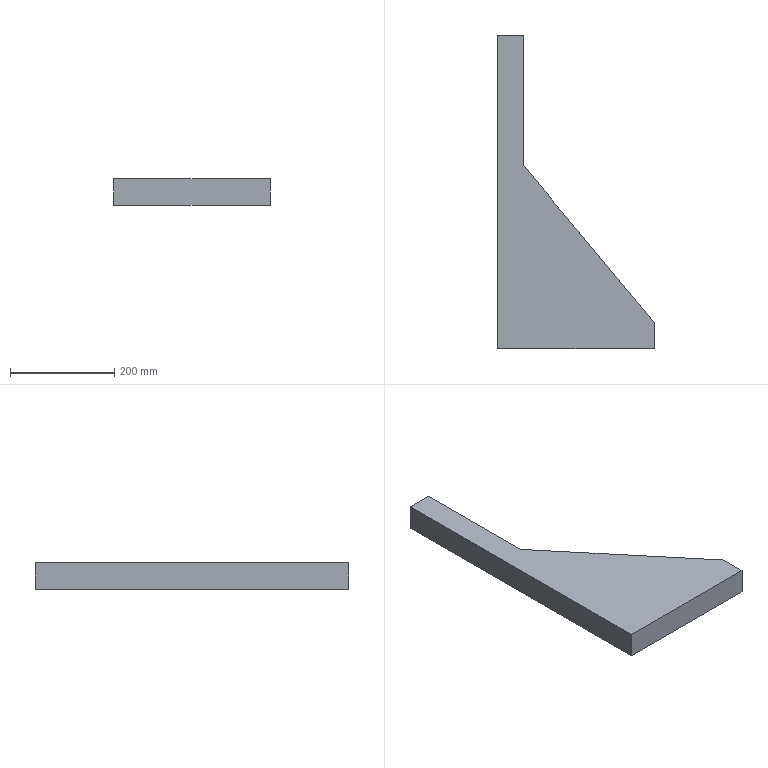Component | SolidWorks | ST60-07-2 | 1 solid | 8 faces | box 300 x 600 x 50 mm | volume 4000000 mm3 | plane 8
build123d program:
from build123d import *

# Parameters (mm, degrees)
BOSS_EXTRUDE1_DEPTH = 50


with BuildPart() as part:
    # Sketch1 → Boss-Extrude1 (new body)
    with BuildSketch(Plane.XY):
        Polygon((0, 300), (0, 0), (600, 0), (600, 50), (350, 50), (50, 300), align=None)
    extrude(amount=BOSS_EXTRUDE1_DEPTH)


solid = part.part

# Placed as in the assembly
solid = solid.moved(Location((277.993, 135.454, -1551.4), (180, 0, -90)))
STEP:
#1=COLOUR_RGB('',0.7922,0.8196,0.9333);
#2=FILL_AREA_STYLE_COLOUR('',#1);
#3=FILL_AREA_STYLE('',(#2));
#4=SURFACE_STYLE_FILL_AREA(#3);
#5=SURFACE_SIDE_STYLE('',(#4));
#6=SURFACE_STYLE_USAGE(.BOTH.,#5);
#7=PRESENTATION_STYLE_ASSIGNMENT((#6));
#8=CARTESIAN_POINT('',(22.756,7.301,-61.079));
#9=VERTEX_POINT('',#8);
#10=CARTESIAN_POINT('',(22.756,5.333,-61.079));
#11=VERTEX_POINT('',#10);
#12=CARTESIAN_POINT('',(22.756,7.301,-61.079));
#13=DIRECTION('',(0.,-1.,0.));
#14=VECTOR('',#13,39.37);
#15=LINE('',#12,#14);
#16=EDGE_CURVE('',#9,#11,#15,.T.);
#17=ORIENTED_EDGE('',*,*,#16,.T.);
#18=CARTESIAN_POINT('',(22.756,5.333,-63.047));
#19=VERTEX_POINT('',#18);
#20=CARTESIAN_POINT('',(22.756,5.333,-63.047));
#21=DIRECTION('',(0.,0.,1.));
#22=VECTOR('',#21,39.37);
#23=LINE('',#20,#22);
#24=EDGE_CURVE('',#19,#11,#23,.T.);
#25=ORIENTED_EDGE('',*,*,#24,.F.);
#26=CARTESIAN_POINT('',(22.756,7.301,-63.047));
#27=VERTEX_POINT('',#26);
#28=CARTESIAN_POINT('',(22.756,7.301,-63.047));
#29=DIRECTION('',(0.,-1.,0.));
#30=VECTOR('',#29,39.37);
#31=LINE('',#28,#30);
#32=EDGE_CURVE('',#27,#19,#31,.T.);
#33=ORIENTED_EDGE('',*,*,#32,.F.);
#34=CARTESIAN_POINT('',(22.756,7.301,-63.047));
#35=DIRECTION('',(0.,0.,1.));
#36=VECTOR('',#35,39.37);
#37=LINE('',#34,#36);
#38=EDGE_CURVE('',#27,#9,#37,.T.);
#39=ORIENTED_EDGE('',*,*,#38,.T.);
#40=EDGE_LOOP('',(#17,#25,#33,#39));
#41=FACE_OUTER_BOUND('',#40,.T.);
#42=CARTESIAN_POINT('',(22.756,7.301,-63.047));
#43=DIRECTION('',(-1.,-0.,0.));
#44=DIRECTION('',(0.,0.,1.));
#45=AXIS2_PLACEMENT_3D('',#42,#43,#44);
#46=PLANE('',#45);
#47=ADVANCED_FACE('',(#41),#46,.F.);
#48=CARTESIAN_POINT('',(10.945,5.333,-61.079));
#49=VERTEX_POINT('',#48);
#50=CARTESIAN_POINT('',(22.756,5.333,-61.079));
#51=DIRECTION('',(-1.,-0.,0.));
#52=VECTOR('',#51,39.37);
#53=LINE('',#50,#52);
#54=EDGE_CURVE('',#11,#49,#53,.T.);
#55=ORIENTED_EDGE('',*,*,#54,.T.);
#56=CARTESIAN_POINT('',(10.945,5.333,-63.047));
#57=VERTEX_POINT('',#56);
#58=CARTESIAN_POINT('',(10.945,5.333,-63.047));
#59=DIRECTION('',(0.,0.,1.));
#60=VECTOR('',#59,39.37);
#61=LINE('',#58,#60);
#62=EDGE_CURVE('',#57,#49,#61,.T.);
#63=ORIENTED_EDGE('',*,*,#62,.F.);
#64=CARTESIAN_POINT('',(22.756,5.333,-63.047));
#65=DIRECTION('',(-1.,-0.,0.));
#66=VECTOR('',#65,39.37);
#67=LINE('',#64,#66);
#68=EDGE_CURVE('',#19,#57,#67,.T.);
#69=ORIENTED_EDGE('',*,*,#68,.F.);
#70=ORIENTED_EDGE('',*,*,#24,.T.);
#71=EDGE_LOOP('',(#55,#63,#69,#70));
#72=FACE_OUTER_BOUND('',#71,.T.);
#73=CARTESIAN_POINT('',(22.756,5.333,-63.047));
#74=DIRECTION('',(-0.,1.,-0.));
#75=DIRECTION('',(1.,0.,-0.));
#76=AXIS2_PLACEMENT_3D('',#73,#74,#75);
#77=PLANE('',#76);
#78=ADVANCED_FACE('',(#72),#77,.F.);
#79=CARTESIAN_POINT('',(10.945,28.955,-61.079));
#80=VERTEX_POINT('',#79);
#81=CARTESIAN_POINT('',(10.945,5.333,-61.079));
#82=DIRECTION('',(-0.,1.,-0.));
#83=VECTOR('',#82,39.37);
#84=LINE('',#81,#83);
#85=EDGE_CURVE('',#49,#80,#84,.T.);
#86=ORIENTED_EDGE('',*,*,#85,.T.);
#87=CARTESIAN_POINT('',(10.945,28.955,-63.047));
#88=VERTEX_POINT('',#87);
#89=CARTESIAN_POINT('',(10.945,28.955,-63.047));
#90=DIRECTION('',(0.,0.,1.));
#91=VECTOR('',#90,39.37);
#92=LINE('',#89,#91);
#93=EDGE_CURVE('',#88,#80,#92,.T.);
#94=ORIENTED_EDGE('',*,*,#93,.F.);
#95=CARTESIAN_POINT('',(10.945,5.333,-63.047));
#96=DIRECTION('',(-0.,1.,-0.));
#97=VECTOR('',#96,39.37);
#98=LINE('',#95,#97);
#99=EDGE_CURVE('',#57,#88,#98,.T.);
#100=ORIENTED_EDGE('',*,*,#99,.F.);
#101=ORIENTED_EDGE('',*,*,#62,.T.);
#102=EDGE_LOOP('',(#86,#94,#100,#101));
#103=FACE_OUTER_BOUND('',#102,.T.);
#104=CARTESIAN_POINT('',(10.945,5.333,-63.047));
#105=DIRECTION('',(1.,0.,-0.));
#106=DIRECTION('',(-0.,-0.,-1.));
#107=AXIS2_PLACEMENT_3D('',#104,#105,#106);
#108=PLANE('',#107);
#109=ADVANCED_FACE('',(#103),#108,.F.);
#110=CARTESIAN_POINT('',(12.913,28.955,-61.079));
#111=VERTEX_POINT('',#110);
#112=CARTESIAN_POINT('',(10.945,28.955,-61.079));
#113=DIRECTION('',(1.,0.,-0.));
#114=VECTOR('',#113,39.37);
#115=LINE('',#112,#114);
#116=EDGE_CURVE('',#80,#111,#115,.T.);
#117=ORIENTED_EDGE('',*,*,#116,.T.);
#118=CARTESIAN_POINT('',(12.913,28.955,-63.047));
#119=VERTEX_POINT('',#118);
#120=CARTESIAN_POINT('',(12.913,28.955,-63.047));
#121=DIRECTION('',(0.,0.,1.));
#122=VECTOR('',#121,39.37);
#123=LINE('',#120,#122);
#124=EDGE_CURVE('',#119,#111,#123,.T.);
#125=ORIENTED_EDGE('',*,*,#124,.F.);
#126=CARTESIAN_POINT('',(10.945,28.955,-63.047));
#127=DIRECTION('',(1.,0.,-0.));
#128=VECTOR('',#127,39.37);
#129=LINE('',#126,#128);
#130=EDGE_CURVE('',#88,#119,#129,.T.);
#131=ORIENTED_EDGE('',*,*,#130,.F.);
#132=ORIENTED_EDGE('',*,*,#93,.T.);
#133=EDGE_LOOP('',(#117,#125,#131,#132));
#134=FACE_OUTER_BOUND('',#133,.T.);
#135=CARTESIAN_POINT('',(10.945,28.955,-63.047));
#136=DIRECTION('',(0.,-1.,0.));
#137=DIRECTION('',(-0.,-0.,-1.));
#138=AXIS2_PLACEMENT_3D('',#135,#136,#137);
#139=PLANE('',#138);
#140=ADVANCED_FACE('',(#134),#139,.F.);
#141=CARTESIAN_POINT('',(12.913,19.112,-61.079));
#142=VERTEX_POINT('',#141);
#143=CARTESIAN_POINT('',(12.913,28.955,-61.079));
#144=DIRECTION('',(-0.,-1.,0.));
#145=VECTOR('',#144,39.37);
#146=LINE('',#143,#145);
#147=EDGE_CURVE('',#111,#142,#146,.T.);
#148=ORIENTED_EDGE('',*,*,#147,.T.);
#149=CARTESIAN_POINT('',(12.913,19.112,-63.047));
#150=VERTEX_POINT('',#149);
#151=CARTESIAN_POINT('',(12.913,19.112,-63.047));
#152=DIRECTION('',(0.,0.,1.));
#153=VECTOR('',#152,39.37);
#154=LINE('',#151,#153);
#155=EDGE_CURVE('',#150,#142,#154,.T.);
#156=ORIENTED_EDGE('',*,*,#155,.F.);
#157=CARTESIAN_POINT('',(12.913,28.955,-63.047));
#158=DIRECTION('',(-0.,-1.,0.));
#159=VECTOR('',#158,39.37);
#160=LINE('',#157,#159);
#161=EDGE_CURVE('',#119,#150,#160,.T.);
#162=ORIENTED_EDGE('',*,*,#161,.F.);
#163=ORIENTED_EDGE('',*,*,#124,.T.);
#164=EDGE_LOOP('',(#148,#156,#162,#163));
#165=FACE_OUTER_BOUND('',#164,.T.);
#166=CARTESIAN_POINT('',(12.913,28.955,-63.047));
#167=DIRECTION('',(-1.,0.,0.));
#168=DIRECTION('',(0.,1.,-0.));
#169=AXIS2_PLACEMENT_3D('',#166,#167,#168);
#170=PLANE('',#169);
#171=ADVANCED_FACE('',(#165),#170,.F.);
#172=CARTESIAN_POINT('',(12.913,19.112,-61.079));
#173=DIRECTION('',(0.6402,-0.7682,-0.));
#174=VECTOR('',#173,39.37);
#175=LINE('',#172,#174);
#176=EDGE_CURVE('',#142,#9,#175,.T.);
#177=ORIENTED_EDGE('',*,*,#176,.T.);
#178=ORIENTED_EDGE('',*,*,#38,.F.);
#179=CARTESIAN_POINT('',(12.913,19.112,-63.047));
#180=DIRECTION('',(0.6402,-0.7682,-0.));
#181=VECTOR('',#180,39.37);
#182=LINE('',#179,#181);
#183=EDGE_CURVE('',#150,#27,#182,.T.);
#184=ORIENTED_EDGE('',*,*,#183,.F.);
#185=ORIENTED_EDGE('',*,*,#155,.T.);
#186=EDGE_LOOP('',(#177,#178,#184,#185));
#187=FACE_OUTER_BOUND('',#186,.T.);
#188=CARTESIAN_POINT('',(12.913,19.112,-63.047));
#189=DIRECTION('',(-0.7682,-0.6402,0.));
#190=DIRECTION('',(-0.6402,0.7682,0.));
#191=AXIS2_PLACEMENT_3D('',#188,#189,#190);
#192=PLANE('',#191);
#193=ADVANCED_FACE('',(#187),#192,.F.);
#194=ORIENTED_EDGE('',*,*,#32,.T.);
#195=ORIENTED_EDGE('',*,*,#68,.T.);
#196=ORIENTED_EDGE('',*,*,#99,.T.);
#197=ORIENTED_EDGE('',*,*,#130,.T.);
#198=ORIENTED_EDGE('',*,*,#161,.T.);
#199=ORIENTED_EDGE('',*,*,#183,.T.);
#200=EDGE_LOOP('',(#194,#195,#196,#197,#198,#199));
#201=FACE_OUTER_BOUND('',#200,.T.);
#202=CARTESIAN_POINT('',(10.945,5.333,-63.047));
#203=DIRECTION('',(-0.,-0.,-1.));
#204=DIRECTION('',(-0.,1.,-0.));
#205=AXIS2_PLACEMENT_3D('',#202,#203,#204);
#206=PLANE('',#205);
#207=ADVANCED_FACE('',(#201),#206,.T.);
#208=ORIENTED_EDGE('',*,*,#16,.F.);
#209=ORIENTED_EDGE('',*,*,#176,.F.);
#210=ORIENTED_EDGE('',*,*,#147,.F.);
#211=ORIENTED_EDGE('',*,*,#116,.F.);
#212=ORIENTED_EDGE('',*,*,#85,.F.);
#213=ORIENTED_EDGE('',*,*,#54,.F.);
#214=EDGE_LOOP('',(#208,#209,#210,#211,#212,#213));
#215=FACE_OUTER_BOUND('',#214,.T.);
#216=CARTESIAN_POINT('',(10.945,5.333,-61.079));
#217=DIRECTION('',(-0.,-0.,-1.));
#218=DIRECTION('',(-0.,1.,-0.));
#219=AXIS2_PLACEMENT_3D('',#216,#217,#218);
#220=PLANE('',#219);
#221=ADVANCED_FACE('',(#215),#220,.F.);
#222=CLOSED_SHELL('',(#47,#78,#109,#140,#171,#193,#207,#221));
#223=MANIFOLD_SOLID_BREP('',#222);
#224=STYLED_ITEM('',(#7),#223);
#225=(LENGTH_UNIT()NAMED_UNIT(*)SI_UNIT($,.METRE.));
#226=LENGTH_MEASURE_WITH_UNIT(LENGTH_MEASURE(0.0254),#225);
#227=DIMENSIONAL_EXPONENTS(1.,0.,0.,0.,0.,0.,0.);
#228=(CONVERSION_BASED_UNIT('',#226)LENGTH_UNIT()NAMED_UNIT(#227));
#229=UNCERTAINTY_MEASURE_WITH_UNIT(LENGTH_MEASURE(0.00001),#228,'','');
#230=(NAMED_UNIT(*)PLANE_ANGLE_UNIT()SI_UNIT($,.RADIAN.));
#231=(NAMED_UNIT(*)SI_UNIT($,.STERADIAN.)SOLID_ANGLE_UNIT());
#232=(GEOMETRIC_REPRESENTATION_CONTEXT(3)GLOBAL_UNCERTAINTY_ASSIGNED_CONTEXT((#229))GLOBAL_UNIT_ASSIGNED_CONTEXT((#228,#230,#231))REPRESENTATION_CONTEXT('',''));
#233=MECHANICAL_DESIGN_GEOMETRIC_PRESENTATION_REPRESENTATION('',(#224),#232);
#234=PRESENTATION_LAYER_ASSIGNMENT('','',(#224));
#235=CARTESIAN_POINT('',(0.,0.,0.));
#236=DIRECTION('',(0.,0.,1.));
#237=DIRECTION('',(1.,0.,0.));
#238=AXIS2_PLACEMENT_3D('',#235,#236,#237);
#239=(LENGTH_UNIT()NAMED_UNIT(*)SI_UNIT($,.METRE.));
#240=LENGTH_MEASURE_WITH_UNIT(LENGTH_MEASURE(0.0254),#239);
#241=DIMENSIONAL_EXPONENTS(1.,0.,0.,0.,0.,0.,0.);
#242=(CONVERSION_BASED_UNIT('',#240)LENGTH_UNIT()NAMED_UNIT(#241));
#243=UNCERTAINTY_MEASURE_WITH_UNIT(LENGTH_MEASURE(0.00001),#242,'','');
#244=(NAMED_UNIT(*)PLANE_ANGLE_UNIT()SI_UNIT($,.RADIAN.));
#245=(NAMED_UNIT(*)SI_UNIT($,.STERADIAN.)SOLID_ANGLE_UNIT());
#246=(GEOMETRIC_REPRESENTATION_CONTEXT(3)GLOBAL_UNCERTAINTY_ASSIGNED_CONTEXT((#243))GLOBAL_UNIT_ASSIGNED_CONTEXT((#242,#244,#245))REPRESENTATION_CONTEXT('',''));
#247=ADVANCED_BREP_SHAPE_REPRESENTATION('',(#223,#238),#246);